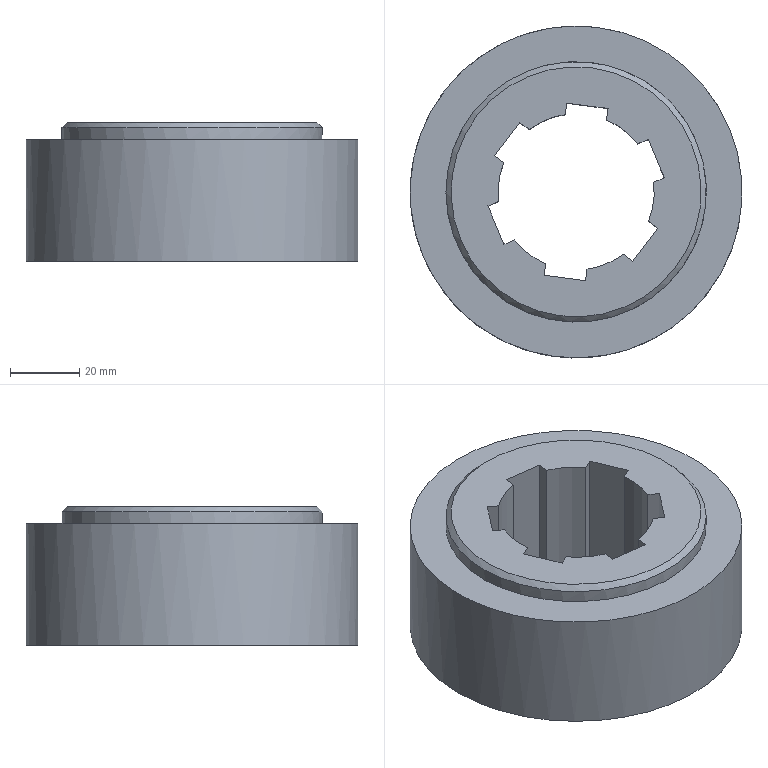Component | NX | ZHOUV4 | 1 solid | 30 faces | volume 201462 mm3 | plane 21 | cylinder 8 | cone 1 | commonest cylinder face diameters 45 x6 95.604 x1 75 x1